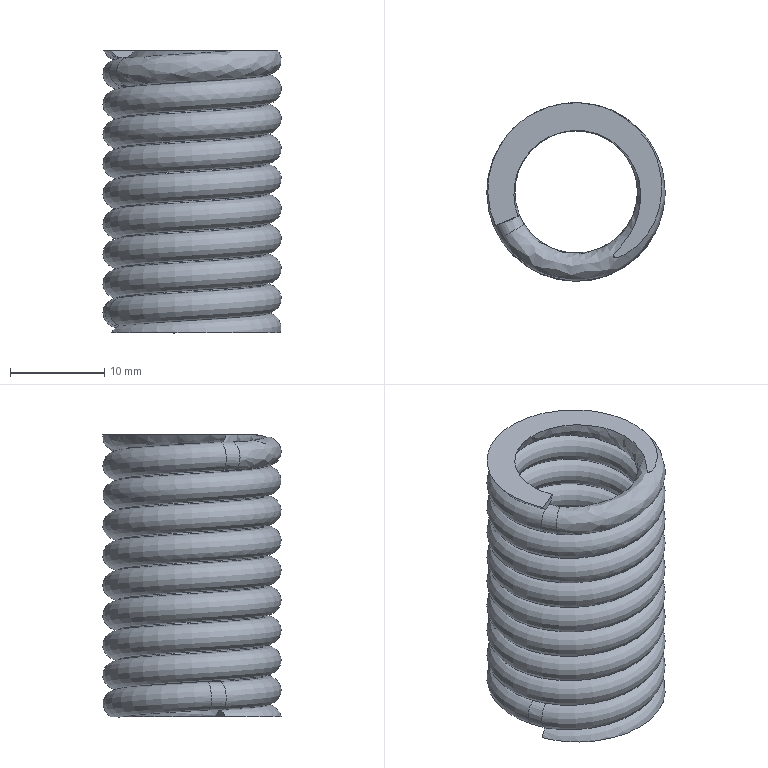Component | NX | SPRING_CYLINDER_COMPRESSION_1 | 1 solid | 9 faces | volume 3353 mm3 | spline 5 | plane 4